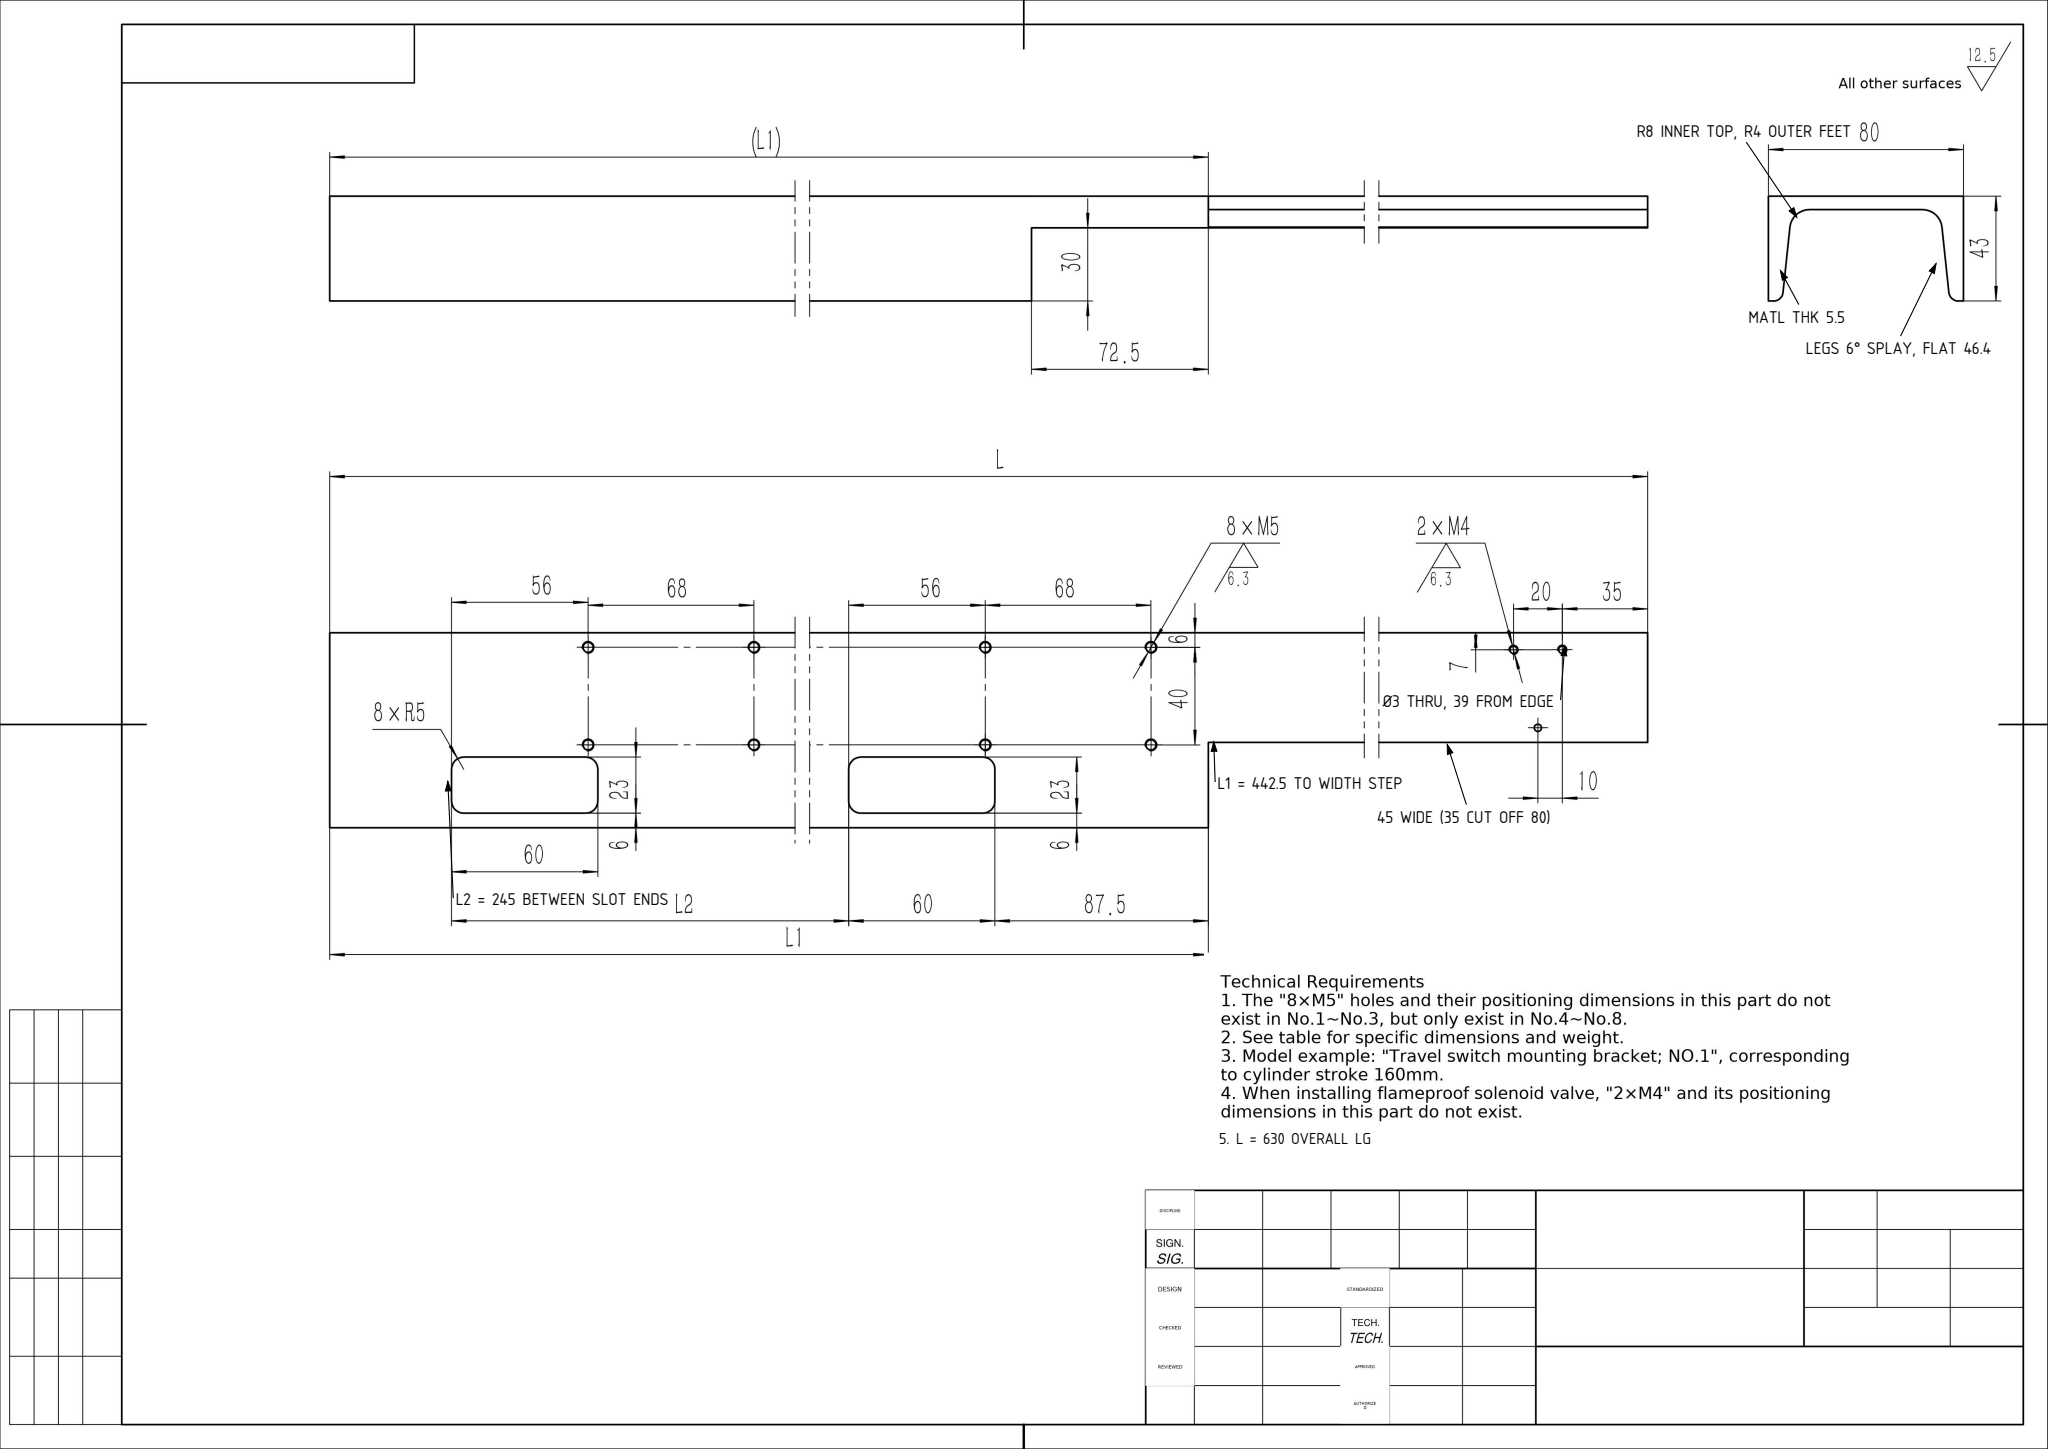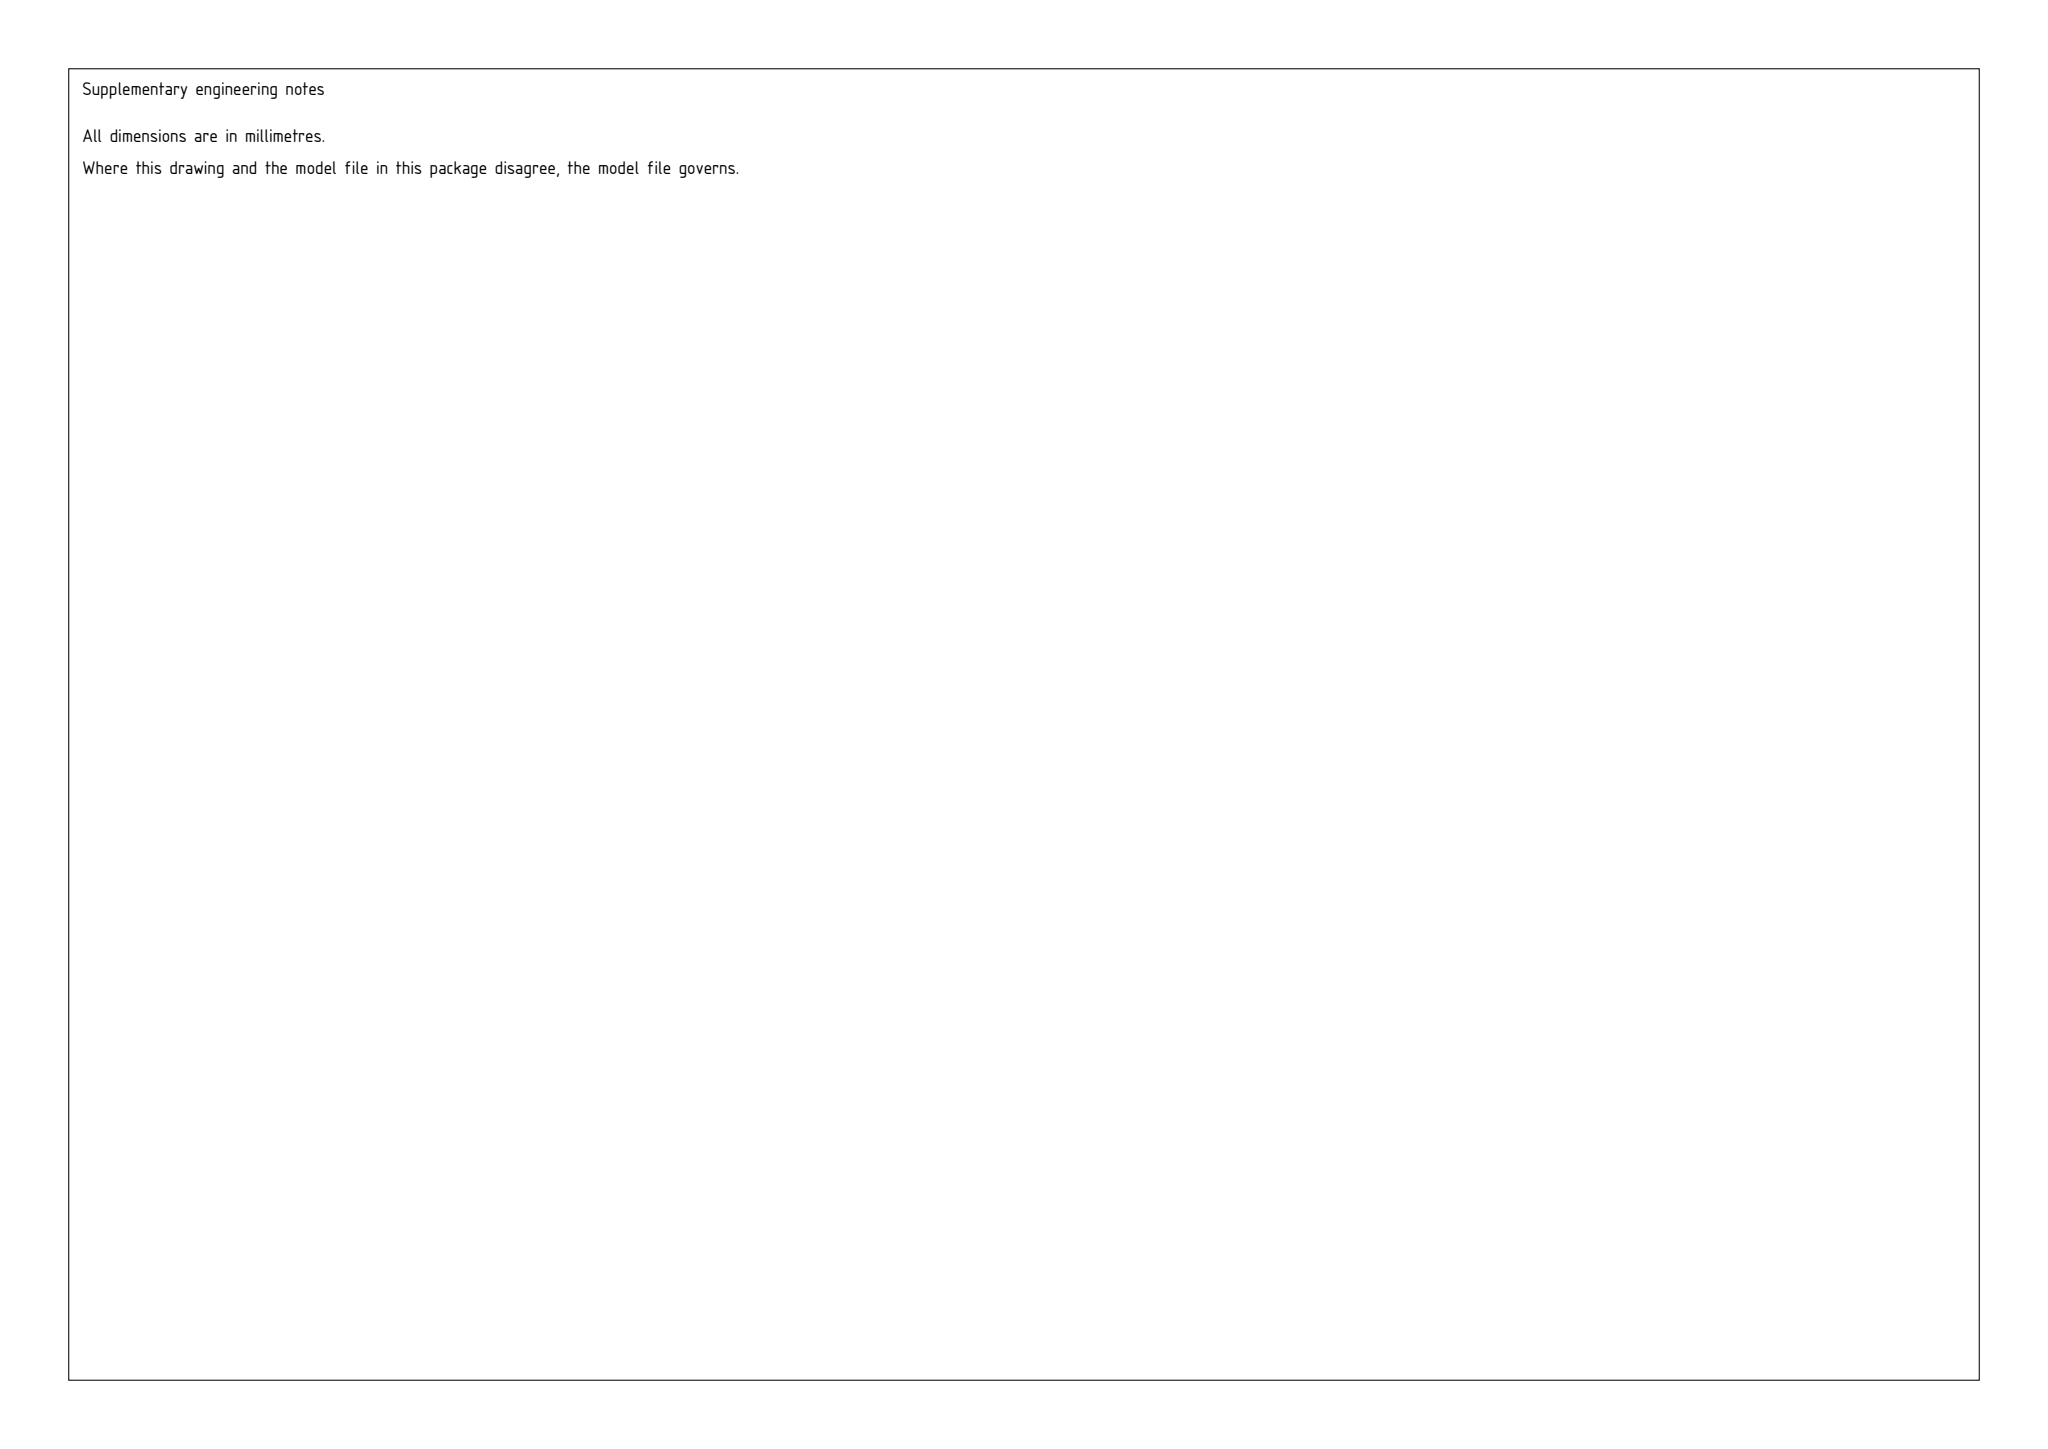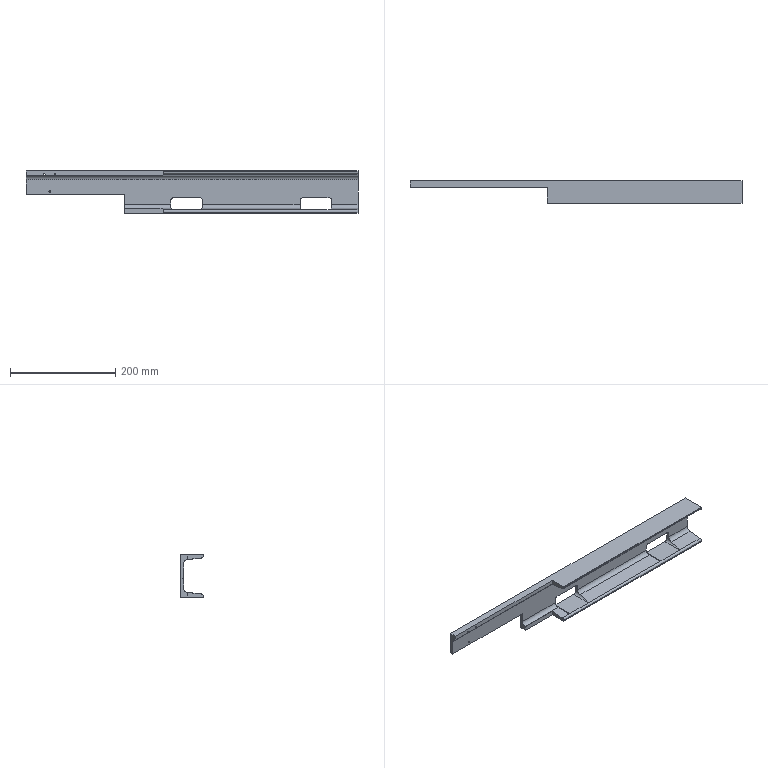Part | SolidWorks | mm | 1 solid | 46 faces | box 630 x 43 x 80 mm | volume 461306 mm3 | plane 26 | cylinder 20 | commonest cylinder face diameters 10 x8 3 x6 16 x4 8 x2
Drawing notes:
L = 630 OVERALL LG | from the solid: bbox_xyz x-extent = 630.0
L1 = 442.5, END FACE TO WIDTH STEP (STEP 72.5 PER TOP VIEW) | from the solid: x-plane 187.5 vs end face x=630 -> 442.5; web step plane x=260 -> 260-187.5=72.5
NARROW SECT BEYOND STEP 45 WIDE (35 CUT OFF 80) | from the solid: z planes 0, 35, 80 -> 80-35=45 wide; step at x=187.5
MATL THK 5.5 THRUOUT CHANNEL SECT | from the solid: y-planes 37.5 and 43.0 -> 5.5; thru-hole cyl length 5.5
FORM BENDS: R8 INNER AT TOP, R4 OUTER AT FEET | from the solid: dia 16 cyls axis x at y=29.5 (z=16.78/63.22) = R8; dia 8 cyls axis x at y=4 (z=2.03/77.97) = R4
LEGS SPLAY 6 DEG FROM VERT; INNER TOP FLAT 46.4 WIDE | from the solid: Inclined leg faces: angle_to_xyz_axes [90,84,6] with bbox size [630, 26.8, 2.8] -> atan(2.8/26.8) = 6 deg from vertical (arc_deg 84 on the R8/R4 bend cylinders confirms); inner top plane y=37.5 spans z 16.8-63.2 = 46.4 wide
L2 = 245 BETWEEN SLOT ENDS; NEAREST SLOT END 55 FROM PART END | from the solid: Slots (R5 ends, dia 10 arcs) occupy x 280-330 and x 525-575; 575-330 = 245 between inner slot ends; bbox x = 630 so nearest slot end is 630-575 = 55 from the end face
UNDIM'D HOLE: Ø3 THRU TOP FLANGE, 39 FROM EDGE | from the solid: dia 3.0 cyl axis y at x=45, z=41, length 5.5 = web thk; 80-41=39 from same edge as 2 x M4 (z=73)